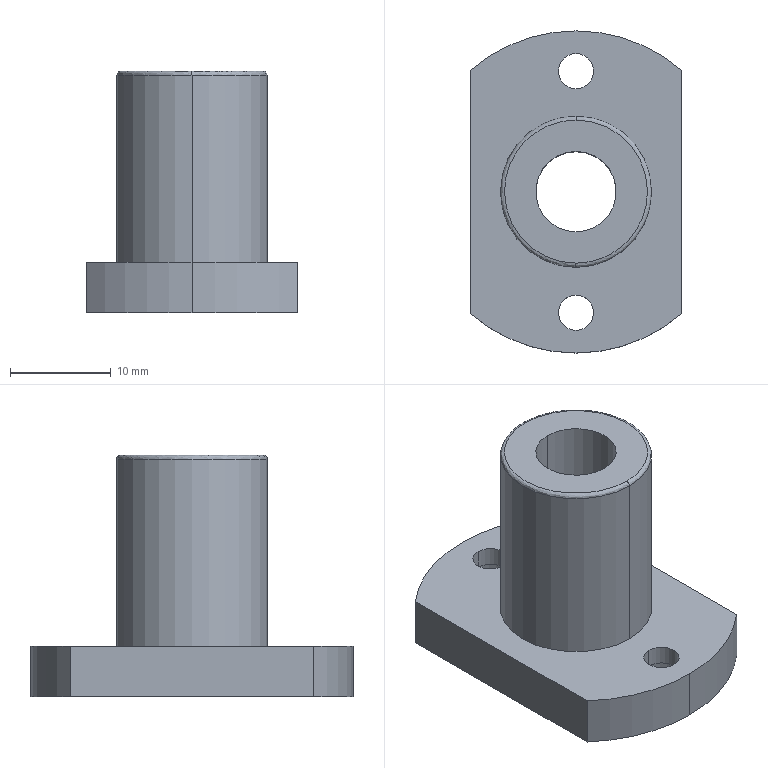Component | SolidWorks | 170423A4-LME21-d8-1 | 1 solid | 24 faces | box 21 x 32 x 24 mm | volume 5038 mm3 | cylinder 15 | plane 7 | spline 2 | commonest cylinder face diameters 3.5 x4 6 x4 32 x3 15 x2 8 x2
STEP:
#1=CARTESIAN_POINT('',(-1.745,-1.815,0.6506));
#2=VERTEX_POINT('',#1);
#3=CARTESIAN_POINT('',(-1.745,-1.225,0.6506));
#4=VERTEX_POINT('',#3);
#5=CARTESIAN_POINT('',(-1.745,-1.52,0.6506));
#6=DIRECTION('',(0.,-0.,-1.));
#7=DIRECTION('',(0.,-1.,0.));
#8=AXIS2_PLACEMENT_3D('',#5,#6,#7);
#9=CIRCLE('',#8,0.2953);
#10=EDGE_CURVE('',#2,#4,#9,.T.);
#11=ORIENTED_EDGE('',*,*,#10,.F.);
#12=CARTESIAN_POINT('',(-1.745,-1.8,0.6664));
#13=VERTEX_POINT('',#12);
#14=CARTESIAN_POINT('',(-1.745,-1.8,0.6506));
#15=DIRECTION('',(-1.,-0.,-0.));
#16=DIRECTION('',(0.,-1.,0.));
#17=AXIS2_PLACEMENT_3D('',#14,#15,#16);
#18=CIRCLE('',#17,0.01575);
#19=EDGE_CURVE('',#2,#13,#18,.T.);
#20=ORIENTED_EDGE('',*,*,#19,.T.);
#21=CARTESIAN_POINT('',(-1.745,-1.241,0.6664));
#22=VERTEX_POINT('',#21);
#23=CARTESIAN_POINT('',(-1.745,-1.8,0.6664));
#24=CARTESIAN_POINT('',(-2.304,-1.8,0.6664));
#25=CARTESIAN_POINT('',(-2.304,-1.241,0.6664));
#26=CARTESIAN_POINT('',(-1.745,-1.241,0.6664));
#27=(BOUNDED_CURVE()B_SPLINE_CURVE(3,(#23,#24,#25,#26),.UNSPECIFIED.,.F.,.F.)B_SPLINE_CURVE_WITH_KNOTS((4,4),(0.5,1.),.UNSPECIFIED.)CURVE()GEOMETRIC_REPRESENTATION_ITEM()RATIONAL_B_SPLINE_CURVE((1.,0.3333,0.3333,1.))REPRESENTATION_ITEM(''));
#28=EDGE_CURVE('',#13,#22,#27,.T.);
#29=ORIENTED_EDGE('',*,*,#28,.T.);
#30=CARTESIAN_POINT('',(-1.745,-1.241,0.6506));
#31=DIRECTION('',(1.,0.,0.));
#32=DIRECTION('',(0.,1.,0.));
#33=AXIS2_PLACEMENT_3D('',#30,#31,#32);
#34=CIRCLE('',#33,0.01575);
#35=EDGE_CURVE('',#4,#22,#34,.T.);
#36=ORIENTED_EDGE('',*,*,#35,.F.);
#37=EDGE_LOOP('',(#11,#20,#29,#36));
#38=FACE_OUTER_BOUND('',#37,.T.);
#39=CARTESIAN_POINT('',(-1.745,-1.815,0.6506));
#40=CARTESIAN_POINT('',(-2.335,-1.815,0.6506));
#41=CARTESIAN_POINT('',(-2.335,-1.225,0.6506));
#42=CARTESIAN_POINT('',(-1.745,-1.225,0.6506));
#43=CARTESIAN_POINT('',(-1.745,-1.815,0.6599));
#44=CARTESIAN_POINT('',(-2.335,-1.815,0.6599));
#45=CARTESIAN_POINT('',(-2.335,-1.225,0.6599));
#46=CARTESIAN_POINT('',(-1.745,-1.225,0.6599));
#47=CARTESIAN_POINT('',(-1.745,-1.809,0.6664));
#48=CARTESIAN_POINT('',(-2.322,-1.809,0.6664));
#49=CARTESIAN_POINT('',(-2.322,-1.231,0.6664));
#50=CARTESIAN_POINT('',(-1.745,-1.231,0.6664));
#51=CARTESIAN_POINT('',(-1.745,-1.8,0.6664));
#52=CARTESIAN_POINT('',(-2.304,-1.8,0.6664));
#53=CARTESIAN_POINT('',(-2.304,-1.241,0.6664));
#54=CARTESIAN_POINT('',(-1.745,-1.241,0.6664));
#55=(BOUNDED_SURFACE()B_SPLINE_SURFACE(3,3,((#39,#40,#41,#42),(#43,#44,#45,#46),(#47,#48,#49,#50),(#51,#52,#53,#54)),.UNSPECIFIED.,.F.,.F.,.F.)B_SPLINE_SURFACE_WITH_KNOTS((4,4),(4,4),(0.,1.),(0.,1.),.UNSPECIFIED.)GEOMETRIC_REPRESENTATION_ITEM()RATIONAL_B_SPLINE_SURFACE(((1.,0.3333,0.3333,1.),(0.8047,0.2682,0.2682,0.8047),(0.8047,0.2682,0.2682,0.8047),(1.,0.3333,0.3333,1.)))REPRESENTATION_ITEM('')SURFACE());
#56=ADVANCED_FACE('',(#38),#55,.T.);
#57=CARTESIAN_POINT('',(-1.745,-1.815,-0.08165));
#58=VERTEX_POINT('',#57);
#59=CARTESIAN_POINT('',(-1.745,-1.225,-0.08165));
#60=VERTEX_POINT('',#59);
#61=CARTESIAN_POINT('',(-1.745,-1.52,-0.08165));
#62=DIRECTION('',(-0.,0.,1.));
#63=DIRECTION('',(0.,-1.,0.));
#64=AXIS2_PLACEMENT_3D('',#61,#62,#63);
#65=CIRCLE('',#64,0.2953);
#66=EDGE_CURVE('',#58,#60,#65,.T.);
#67=ORIENTED_EDGE('',*,*,#66,.T.);
#68=CARTESIAN_POINT('',(-1.745,-1.225,-0.2785));
#69=DIRECTION('',(-0.,0.,1.));
#70=VECTOR('',#69,39.37);
#71=LINE('',#68,#70);
#72=EDGE_CURVE('',#60,#4,#71,.T.);
#73=ORIENTED_EDGE('',*,*,#72,.T.);
#74=CARTESIAN_POINT('',(-1.745,-1.52,0.6506));
#75=DIRECTION('',(0.,-0.,-1.));
#76=DIRECTION('',(0.,-1.,0.));
#77=AXIS2_PLACEMENT_3D('',#74,#75,#76);
#78=CIRCLE('',#77,0.2953);
#79=EDGE_CURVE('',#4,#2,#78,.T.);
#80=ORIENTED_EDGE('',*,*,#79,.T.);
#81=CARTESIAN_POINT('',(-1.745,-1.815,-0.2785));
#82=DIRECTION('',(-0.,0.,1.));
#83=VECTOR('',#82,39.37);
#84=LINE('',#81,#83);
#85=EDGE_CURVE('',#58,#2,#84,.T.);
#86=ORIENTED_EDGE('',*,*,#85,.F.);
#87=EDGE_LOOP('',(#67,#73,#80,#86));
#88=FACE_OUTER_BOUND('',#87,.T.);
#89=CARTESIAN_POINT('',(-1.745,-1.52,-0.2785));
#90=DIRECTION('',(-0.,0.,1.));
#91=DIRECTION('',(0.,-1.,0.));
#92=AXIS2_PLACEMENT_3D('',#89,#90,#91);
#93=CYLINDRICAL_SURFACE('',#92,0.2953);
#94=ADVANCED_FACE('',(#88),#93,.T.);
#95=CARTESIAN_POINT('',(-1.745,-2.061,-0.08165));
#96=VERTEX_POINT('',#95);
#97=CARTESIAN_POINT('',(-1.745,-1.924,-0.08165));
#98=VERTEX_POINT('',#97);
#99=CARTESIAN_POINT('',(-1.745,-1.993,-0.08165));
#100=DIRECTION('',(0.,0.,-1.));
#101=DIRECTION('',(0.,1.,-0.));
#102=AXIS2_PLACEMENT_3D('',#99,#100,#101);
#103=CIRCLE('',#102,0.0689);
#104=EDGE_CURVE('',#96,#98,#103,.T.);
#105=ORIENTED_EDGE('',*,*,#104,.F.);
#106=CARTESIAN_POINT('',(-1.745,-2.061,-0.1564));
#107=VERTEX_POINT('',#106);
#108=CARTESIAN_POINT('',(-1.745,-2.061,-0.08165));
#109=DIRECTION('',(0.,0.,-1.));
#110=VECTOR('',#109,39.37);
#111=LINE('',#108,#110);
#112=EDGE_CURVE('',#96,#107,#111,.T.);
#113=ORIENTED_EDGE('',*,*,#112,.T.);
#114=CARTESIAN_POINT('',(-1.745,-1.924,-0.1564));
#115=VERTEX_POINT('',#114);
#116=CARTESIAN_POINT('',(-1.745,-1.993,-0.1564));
#117=DIRECTION('',(-0.,-0.,1.));
#118=DIRECTION('',(0.,1.,0.));
#119=AXIS2_PLACEMENT_3D('',#116,#117,#118);
#120=CIRCLE('',#119,0.0689);
#121=EDGE_CURVE('',#115,#107,#120,.T.);
#122=ORIENTED_EDGE('',*,*,#121,.F.);
#123=CARTESIAN_POINT('',(-1.745,-1.924,-0.08165));
#124=DIRECTION('',(0.,0.,-1.));
#125=VECTOR('',#124,39.37);
#126=LINE('',#123,#125);
#127=EDGE_CURVE('',#98,#115,#126,.T.);
#128=ORIENTED_EDGE('',*,*,#127,.F.);
#129=EDGE_LOOP('',(#105,#113,#122,#128));
#130=FACE_OUTER_BOUND('',#129,.T.);
#131=CARTESIAN_POINT('',(-1.745,-1.993,-0.08165));
#132=DIRECTION('',(0.,0.,-1.));
#133=DIRECTION('',(0.,1.,-0.));
#134=AXIS2_PLACEMENT_3D('',#131,#132,#133);
#135=CYLINDRICAL_SURFACE('',#134,0.0689);
#136=ADVANCED_FACE('',(#130),#135,.F.);
#137=CARTESIAN_POINT('',(-2.158,-1.995,-0.2785));
#138=VERTEX_POINT('',#137);
#139=CARTESIAN_POINT('',(-1.745,-2.15,-0.2785));
#140=VERTEX_POINT('',#139);
#141=CARTESIAN_POINT('',(-1.745,-1.52,-0.2785));
#142=DIRECTION('',(-0.,-0.,1.));
#143=DIRECTION('',(0.,-1.,0.));
#144=AXIS2_PLACEMENT_3D('',#141,#142,#143);
#145=CIRCLE('',#144,0.6299);
#146=EDGE_CURVE('',#138,#140,#145,.T.);
#147=ORIENTED_EDGE('',*,*,#146,.T.);
#148=CARTESIAN_POINT('',(-1.745,-2.15,-0.08165));
#149=VERTEX_POINT('',#148);
#150=CARTESIAN_POINT('',(-1.745,-2.15,-0.08165));
#151=DIRECTION('',(-0.,-0.,1.));
#152=VECTOR('',#151,39.37);
#153=LINE('',#150,#152);
#154=EDGE_CURVE('',#140,#149,#153,.T.);
#155=ORIENTED_EDGE('',*,*,#154,.T.);
#156=CARTESIAN_POINT('',(-2.158,-1.995,-0.08165));
#157=VERTEX_POINT('',#156);
#158=CARTESIAN_POINT('',(-1.745,-1.52,-0.08165));
#159=DIRECTION('',(-0.,-0.,1.));
#160=DIRECTION('',(0.,-1.,0.));
#161=AXIS2_PLACEMENT_3D('',#158,#159,#160);
#162=CIRCLE('',#161,0.6299);
#163=EDGE_CURVE('',#157,#149,#162,.T.);
#164=ORIENTED_EDGE('',*,*,#163,.F.);
#165=CARTESIAN_POINT('',(-2.158,-1.995,-0.08165));
#166=DIRECTION('',(0.,0.,-1.));
#167=VECTOR('',#166,39.37);
#168=LINE('',#165,#167);
#169=EDGE_CURVE('',#157,#138,#168,.T.);
#170=ORIENTED_EDGE('',*,*,#169,.T.);
#171=EDGE_LOOP('',(#147,#155,#164,#170));
#172=FACE_OUTER_BOUND('',#171,.T.);
#173=CARTESIAN_POINT('',(-1.745,-1.52,-0.08165));
#174=DIRECTION('',(-0.,-0.,1.));
#175=DIRECTION('',(0.,-1.,0.));
#176=AXIS2_PLACEMENT_3D('',#173,#174,#175);
#177=CYLINDRICAL_SURFACE('',#176,0.6299);
#178=ADVANCED_FACE('',(#172),#177,.T.);
#179=CARTESIAN_POINT('',(-1.745,-0.9788,-0.1564));
#180=VERTEX_POINT('',#179);
#181=CARTESIAN_POINT('',(-1.745,-1.117,-0.1564));
#182=VERTEX_POINT('',#181);
#183=CARTESIAN_POINT('',(-1.745,-1.048,-0.1564));
#184=DIRECTION('',(-0.,-0.,1.));
#185=DIRECTION('',(0.,-1.,0.));
#186=AXIS2_PLACEMENT_3D('',#183,#184,#185);
#187=CIRCLE('',#186,0.0689);
#188=EDGE_CURVE('',#180,#182,#187,.T.);
#189=ORIENTED_EDGE('',*,*,#188,.F.);
#190=CARTESIAN_POINT('',(-1.745,-0.9788,-0.08165));
#191=VERTEX_POINT('',#190);
#192=CARTESIAN_POINT('',(-1.745,-0.9788,-0.2785));
#193=DIRECTION('',(-0.,-0.,1.));
#194=VECTOR('',#193,39.37);
#195=LINE('',#192,#194);
#196=EDGE_CURVE('',#180,#191,#195,.T.);
#197=ORIENTED_EDGE('',*,*,#196,.T.);
#198=CARTESIAN_POINT('',(-1.745,-1.117,-0.08165));
#199=VERTEX_POINT('',#198);
#200=CARTESIAN_POINT('',(-1.745,-1.048,-0.08165));
#201=DIRECTION('',(0.,0.,-1.));
#202=DIRECTION('',(0.,-1.,0.));
#203=AXIS2_PLACEMENT_3D('',#200,#201,#202);
#204=CIRCLE('',#203,0.0689);
#205=EDGE_CURVE('',#199,#191,#204,.T.);
#206=ORIENTED_EDGE('',*,*,#205,.F.);
#207=CARTESIAN_POINT('',(-1.745,-1.117,-0.2785));
#208=DIRECTION('',(-0.,-0.,1.));
#209=VECTOR('',#208,39.37);
#210=LINE('',#207,#209);
#211=EDGE_CURVE('',#182,#199,#210,.T.);
#212=ORIENTED_EDGE('',*,*,#211,.F.);
#213=EDGE_LOOP('',(#189,#197,#206,#212));
#214=FACE_OUTER_BOUND('',#213,.T.);
#215=CARTESIAN_POINT('',(-1.745,-1.048,-0.2785));
#216=DIRECTION('',(-0.,-0.,1.));
#217=DIRECTION('',(0.,-1.,0.));
#218=AXIS2_PLACEMENT_3D('',#215,#216,#217);
#219=CYLINDRICAL_SURFACE('',#218,0.0689);
#220=ADVANCED_FACE('',(#214),#219,.F.);
#221=CARTESIAN_POINT('',(-1.745,-1.363,-0.2785));
#222=VERTEX_POINT('',#221);
#223=CARTESIAN_POINT('',(-1.745,-1.678,-0.2785));
#224=VERTEX_POINT('',#223);
#225=CARTESIAN_POINT('',(-1.745,-1.52,-0.2785));
#226=DIRECTION('',(-0.,0.,1.));
#227=DIRECTION('',(0.,-1.,0.));
#228=AXIS2_PLACEMENT_3D('',#225,#226,#227);
#229=CIRCLE('',#228,0.1575);
#230=EDGE_CURVE('',#222,#224,#229,.T.);
#231=ORIENTED_EDGE('',*,*,#230,.F.);
#232=CARTESIAN_POINT('',(-1.745,-1.363,0.6664));
#233=VERTEX_POINT('',#232);
#234=CARTESIAN_POINT('',(-1.745,-1.363,-0.2785));
#235=DIRECTION('',(-0.,0.,1.));
#236=VECTOR('',#235,39.37);
#237=LINE('',#234,#236);
#238=EDGE_CURVE('',#222,#233,#237,.T.);
#239=ORIENTED_EDGE('',*,*,#238,.T.);
#240=CARTESIAN_POINT('',(-1.745,-1.678,0.6664));
#241=VERTEX_POINT('',#240);
#242=CARTESIAN_POINT('',(-1.745,-1.52,0.6664));
#243=DIRECTION('',(0.,-0.,-1.));
#244=DIRECTION('',(0.,-1.,0.));
#245=AXIS2_PLACEMENT_3D('',#242,#243,#244);
#246=CIRCLE('',#245,0.1575);
#247=EDGE_CURVE('',#241,#233,#246,.T.);
#248=ORIENTED_EDGE('',*,*,#247,.F.);
#249=CARTESIAN_POINT('',(-1.745,-1.678,-0.2785));
#250=DIRECTION('',(-0.,0.,1.));
#251=VECTOR('',#250,39.37);
#252=LINE('',#249,#251);
#253=EDGE_CURVE('',#224,#241,#252,.T.);
#254=ORIENTED_EDGE('',*,*,#253,.F.);
#255=EDGE_LOOP('',(#231,#239,#248,#254));
#256=FACE_OUTER_BOUND('',#255,.T.);
#257=CARTESIAN_POINT('',(-1.745,-1.52,-0.2785));
#258=DIRECTION('',(-0.,0.,1.));
#259=DIRECTION('',(0.,-1.,0.));
#260=AXIS2_PLACEMENT_3D('',#257,#258,#259);
#261=CYLINDRICAL_SURFACE('',#260,0.1575);
#262=ADVANCED_FACE('',(#256),#261,.F.);
#263=CARTESIAN_POINT('',(-1.745,-2.111,-0.1564));
#264=VERTEX_POINT('',#263);
#265=CARTESIAN_POINT('',(-1.745,-1.874,-0.1564));
#266=VERTEX_POINT('',#265);
#267=CARTESIAN_POINT('',(-1.745,-1.993,-0.1564));
#268=DIRECTION('',(0.,0.,-1.));
#269=DIRECTION('',(0.,1.,-0.));
#270=AXIS2_PLACEMENT_3D('',#267,#268,#269);
#271=CIRCLE('',#270,0.1181);
#272=EDGE_CURVE('',#264,#266,#271,.T.);
#273=ORIENTED_EDGE('',*,*,#272,.F.);
#274=CARTESIAN_POINT('',(-1.745,-2.111,-0.2785));
#275=VERTEX_POINT('',#274);
#276=CARTESIAN_POINT('',(-1.745,-2.111,-0.08165));
#277=DIRECTION('',(0.,0.,-1.));
#278=VECTOR('',#277,39.37);
#279=LINE('',#276,#278);
#280=EDGE_CURVE('',#264,#275,#279,.T.);
#281=ORIENTED_EDGE('',*,*,#280,.T.);
#282=CARTESIAN_POINT('',(-1.745,-1.874,-0.2785));
#283=VERTEX_POINT('',#282);
#284=CARTESIAN_POINT('',(-1.745,-1.993,-0.2785));
#285=DIRECTION('',(-0.,-0.,1.));
#286=DIRECTION('',(0.,1.,-0.));
#287=AXIS2_PLACEMENT_3D('',#284,#285,#286);
#288=CIRCLE('',#287,0.1181);
#289=EDGE_CURVE('',#283,#275,#288,.T.);
#290=ORIENTED_EDGE('',*,*,#289,.F.);
#291=CARTESIAN_POINT('',(-1.745,-1.874,-0.08165));
#292=DIRECTION('',(0.,0.,-1.));
#293=VECTOR('',#292,39.37);
#294=LINE('',#291,#293);
#295=EDGE_CURVE('',#266,#283,#294,.T.);
#296=ORIENTED_EDGE('',*,*,#295,.F.);
#297=EDGE_LOOP('',(#273,#281,#290,#296));
#298=FACE_OUTER_BOUND('',#297,.T.);
#299=CARTESIAN_POINT('',(-1.745,-1.993,-0.08165));
#300=DIRECTION('',(0.,0.,-1.));
#301=DIRECTION('',(0.,1.,-0.));
#302=AXIS2_PLACEMENT_3D('',#299,#300,#301);
#303=CYLINDRICAL_SURFACE('',#302,0.1181);
#304=ADVANCED_FACE('',(#298),#303,.F.);
#305=CARTESIAN_POINT('',(-1.745,-0.9296,-0.2785));
#306=VERTEX_POINT('',#305);
#307=CARTESIAN_POINT('',(-1.745,-1.166,-0.2785));
#308=VERTEX_POINT('',#307);
#309=CARTESIAN_POINT('',(-1.745,-1.048,-0.2785));
#310=DIRECTION('',(-0.,-0.,1.));
#311=DIRECTION('',(0.,-1.,0.));
#312=AXIS2_PLACEMENT_3D('',#309,#310,#311);
#313=CIRCLE('',#312,0.1181);
#314=EDGE_CURVE('',#306,#308,#313,.T.);
#315=ORIENTED_EDGE('',*,*,#314,.F.);
#316=CARTESIAN_POINT('',(-1.745,-0.9296,-0.1564));
#317=VERTEX_POINT('',#316);
#318=CARTESIAN_POINT('',(-1.745,-0.9296,-0.2785));
#319=DIRECTION('',(-0.,-0.,1.));
#320=VECTOR('',#319,39.37);
#321=LINE('',#318,#320);
#322=EDGE_CURVE('',#306,#317,#321,.T.);
#323=ORIENTED_EDGE('',*,*,#322,.T.);
#324=CARTESIAN_POINT('',(-1.745,-1.166,-0.1564));
#325=VERTEX_POINT('',#324);
#326=CARTESIAN_POINT('',(-1.745,-1.048,-0.1564));
#327=DIRECTION('',(0.,0.,-1.));
#328=DIRECTION('',(0.,-1.,0.));
#329=AXIS2_PLACEMENT_3D('',#326,#327,#328);
#330=CIRCLE('',#329,0.1181);
#331=EDGE_CURVE('',#325,#317,#330,.T.);
#332=ORIENTED_EDGE('',*,*,#331,.F.);
#333=CARTESIAN_POINT('',(-1.745,-1.166,-0.2785));
#334=DIRECTION('',(-0.,-0.,1.));
#335=VECTOR('',#334,39.37);
#336=LINE('',#333,#335);
#337=EDGE_CURVE('',#308,#325,#336,.T.);
#338=ORIENTED_EDGE('',*,*,#337,.F.);
#339=EDGE_LOOP('',(#315,#323,#332,#338));
#340=FACE_OUTER_BOUND('',#339,.T.);
#341=CARTESIAN_POINT('',(-1.745,-1.048,-0.2785));
#342=DIRECTION('',(-0.,-0.,1.));
#343=DIRECTION('',(0.,-1.,0.));
#344=AXIS2_PLACEMENT_3D('',#341,#342,#343);
#345=CYLINDRICAL_SURFACE('',#344,0.1181);
#346=ADVANCED_FACE('',(#340),#345,.F.);
#347=ORIENTED_EDGE('',*,*,#72,.F.);
#348=CARTESIAN_POINT('',(-1.745,-1.52,-0.08165));
#349=DIRECTION('',(-0.,0.,1.));
#350=DIRECTION('',(0.,-1.,0.));
#351=AXIS2_PLACEMENT_3D('',#348,#349,#350);
#352=CIRCLE('',#351,0.2953);
#353=EDGE_CURVE('',#60,#58,#352,.T.);
#354=ORIENTED_EDGE('',*,*,#353,.T.);
#355=ORIENTED_EDGE('',*,*,#85,.T.);
#356=ORIENTED_EDGE('',*,*,#10,.T.);
#357=EDGE_LOOP('',(#347,#354,#355,#356));
#358=FACE_OUTER_BOUND('',#357,.T.);
#359=CARTESIAN_POINT('',(-1.745,-1.52,-0.2785));
#360=DIRECTION('',(-0.,0.,1.));
#361=DIRECTION('',(0.,-1.,0.));
#362=AXIS2_PLACEMENT_3D('',#359,#360,#361);
#363=CYLINDRICAL_SURFACE('',#362,0.2953);
#364=ADVANCED_FACE('',(#358),#363,.T.);
#365=CARTESIAN_POINT('',(-1.745,-1.993,-0.08165));
#366=DIRECTION('',(0.,0.,-1.));
#367=DIRECTION('',(0.,1.,-0.));
#368=AXIS2_PLACEMENT_3D('',#365,#366,#367);
#369=CIRCLE('',#368,0.0689);
#370=EDGE_CURVE('',#98,#96,#369,.T.);
#371=ORIENTED_EDGE('',*,*,#370,.T.);
#372=ORIENTED_EDGE('',*,*,#104,.T.);
#373=EDGE_LOOP('',(#371,#372));
#374=FACE_BOUND('',#373,.T.);
#375=CARTESIAN_POINT('',(-2.158,-1.045,-0.08165));
#376=VERTEX_POINT('',#375);
#377=CARTESIAN_POINT('',(-2.158,-1.52,-0.08165));
#378=DIRECTION('',(0.,-1.,0.));
#379=VECTOR('',#378,39.37);
#380=LINE('',#377,#379);
#381=EDGE_CURVE('',#376,#157,#380,.T.);
#382=ORIENTED_EDGE('',*,*,#381,.T.);
#383=ORIENTED_EDGE('',*,*,#163,.T.);
#384=CARTESIAN_POINT('',(-1.331,-1.995,-0.08165));
#385=VERTEX_POINT('',#384);
#386=CARTESIAN_POINT('',(-1.745,-1.52,-0.08165));
#387=DIRECTION('',(-0.,-0.,1.));
#388=DIRECTION('',(0.,-1.,0.));
#389=AXIS2_PLACEMENT_3D('',#386,#387,#388);
#390=CIRCLE('',#389,0.6299);
#391=EDGE_CURVE('',#149,#385,#390,.T.);
#392=ORIENTED_EDGE('',*,*,#391,.T.);
#393=CARTESIAN_POINT('',(-1.331,-1.045,-0.08165));
#394=VERTEX_POINT('',#393);
#395=CARTESIAN_POINT('',(-1.331,-1.52,-0.08165));
#396=DIRECTION('',(-0.,1.,-0.));
#397=VECTOR('',#396,39.37);
#398=LINE('',#395,#397);
#399=EDGE_CURVE('',#385,#394,#398,.T.);
#400=ORIENTED_EDGE('',*,*,#399,.T.);
#401=CARTESIAN_POINT('',(-1.745,-1.52,-0.08165));
#402=DIRECTION('',(-0.,-0.,1.));
#403=DIRECTION('',(0.,-1.,0.));
#404=AXIS2_PLACEMENT_3D('',#401,#402,#403);
#405=CIRCLE('',#404,0.6299);
#406=EDGE_CURVE('',#394,#376,#405,.T.);
#407=ORIENTED_EDGE('',*,*,#406,.T.);
#408=EDGE_LOOP('',(#382,#383,#392,#400,#407));
#409=FACE_OUTER_BOUND('',#408,.T.);
#410=ORIENTED_EDGE('',*,*,#66,.F.);
#411=ORIENTED_EDGE('',*,*,#353,.F.);
#412=EDGE_LOOP('',(#410,#411));
#413=FACE_BOUND('',#412,.T.);
#414=ORIENTED_EDGE('',*,*,#205,.T.);
#415=CARTESIAN_POINT('',(-1.745,-1.048,-0.08165));
#416=DIRECTION('',(0.,0.,-1.));
#417=DIRECTION('',(0.,-1.,0.));
#418=AXIS2_PLACEMENT_3D('',#415,#416,#417);
#419=CIRCLE('',#418,0.0689);
#420=EDGE_CURVE('',#191,#199,#419,.T.);
#421=ORIENTED_EDGE('',*,*,#420,.T.);
#422=EDGE_LOOP('',(#414,#421));
#423=FACE_BOUND('',#422,.T.);
#424=CARTESIAN_POINT('',(-1.745,-1.52,-0.08165));
#425=DIRECTION('',(-0.,0.,1.));
#426=DIRECTION('',(0.,-1.,0.));
#427=AXIS2_PLACEMENT_3D('',#424,#425,#426);
#428=PLANE('',#427);
#429=ADVANCED_FACE('',(#374,#409,#413,#423),#428,.T.);
#430=ORIENTED_EDGE('',*,*,#19,.F.);
#431=ORIENTED_EDGE('',*,*,#79,.F.);
#432=ORIENTED_EDGE('',*,*,#35,.T.);
#433=CARTESIAN_POINT('',(-1.745,-1.241,0.6664));
#434=CARTESIAN_POINT('',(-1.186,-1.241,0.6664));
#435=CARTESIAN_POINT('',(-1.186,-1.8,0.6664));
#436=CARTESIAN_POINT('',(-1.745,-1.8,0.6664));
#437=(BOUNDED_CURVE()B_SPLINE_CURVE(3,(#433,#434,#435,#436),.UNSPECIFIED.,.F.,.F.)B_SPLINE_CURVE_WITH_KNOTS((4,4),(0.,0.5),.UNSPECIFIED.)CURVE()GEOMETRIC_REPRESENTATION_ITEM()RATIONAL_B_SPLINE_CURVE((1.,0.3333,0.3333,1.))REPRESENTATION_ITEM(''));
#438=EDGE_CURVE('',#22,#13,#437,.T.);
#439=ORIENTED_EDGE('',*,*,#438,.T.);
#440=EDGE_LOOP('',(#430,#431,#432,#439));
#441=FACE_OUTER_BOUND('',#440,.T.);
#442=CARTESIAN_POINT('',(-1.745,-1.225,0.6506));
#443=CARTESIAN_POINT('',(-1.154,-1.225,0.6506));
#444=CARTESIAN_POINT('',(-1.154,-1.815,0.6506));
#445=CARTESIAN_POINT('',(-1.745,-1.815,0.6506));
#446=CARTESIAN_POINT('',(-1.745,-1.225,0.6599));
#447=CARTESIAN_POINT('',(-1.154,-1.225,0.6599));
#448=CARTESIAN_POINT('',(-1.154,-1.815,0.6599));
#449=CARTESIAN_POINT('',(-1.745,-1.815,0.6599));
#450=CARTESIAN_POINT('',(-1.745,-1.231,0.6664));
#451=CARTESIAN_POINT('',(-1.167,-1.231,0.6664));
#452=CARTESIAN_POINT('',(-1.167,-1.809,0.6664));
#453=CARTESIAN_POINT('',(-1.745,-1.809,0.6664));
#454=CARTESIAN_POINT('',(-1.745,-1.241,0.6664));
#455=CARTESIAN_POINT('',(-1.186,-1.241,0.6664));
#456=CARTESIAN_POINT('',(-1.186,-1.8,0.6664));
#457=CARTESIAN_POINT('',(-1.745,-1.8,0.6664));
#458=(BOUNDED_SURFACE()B_SPLINE_SURFACE(3,3,((#442,#443,#444,#445),(#446,#447,#448,#449),(#450,#451,#452,#453),(#454,#455,#456,#457)),.UNSPECIFIED.,.F.,.F.,.F.)B_SPLINE_SURFACE_WITH_KNOTS((4,4),(4,4),(0.,1.),(0.,1.),.UNSPECIFIED.)GEOMETRIC_REPRESENTATION_ITEM()RATIONAL_B_SPLINE_SURFACE(((1.,0.3333,0.3333,1.),(0.8047,0.2682,0.2682,0.8047),(0.8047,0.2682,0.2682,0.8047),(1.,0.3333,0.3333,1.)))REPRESENTATION_ITEM('')SURFACE());
#459=ADVANCED_FACE('',(#441),#458,.T.);
#460=ORIENTED_EDGE('',*,*,#112,.F.);
#461=ORIENTED_EDGE('',*,*,#370,.F.);
#462=ORIENTED_EDGE('',*,*,#127,.T.);
#463=CARTESIAN_POINT('',(-1.745,-1.993,-0.1564));
#464=DIRECTION('',(-0.,-0.,1.));
#465=DIRECTION('',(0.,1.,0.));
#466=AXIS2_PLACEMENT_3D('',#463,#464,#465);
#467=CIRCLE('',#466,0.0689);
#468=EDGE_CURVE('',#107,#115,#467,.T.);
#469=ORIENTED_EDGE('',*,*,#468,.F.);
#470=EDGE_LOOP('',(#460,#461,#462,#469));
#471=FACE_OUTER_BOUND('',#470,.T.);
#472=CARTESIAN_POINT('',(-1.745,-1.993,-0.08165));
#473=DIRECTION('',(0.,0.,-1.));
#474=DIRECTION('',(0.,1.,-0.));
#475=AXIS2_PLACEMENT_3D('',#472,#473,#474);
#476=CYLINDRICAL_SURFACE('',#475,0.0689);
#477=ADVANCED_FACE('',(#471),#476,.F.);
#478=ORIENTED_EDGE('',*,*,#154,.F.);
#479=CARTESIAN_POINT('',(-1.331,-1.995,-0.2785));
#480=VERTEX_POINT('',#479);
#481=CARTESIAN_POINT('',(-1.745,-1.52,-0.2785));
#482=DIRECTION('',(-0.,-0.,1.));
#483=DIRECTION('',(0.,-1.,0.));
#484=AXIS2_PLACEMENT_3D('',#481,#482,#483);
#485=CIRCLE('',#484,0.6299);
#486=EDGE_CURVE('',#140,#480,#485,.T.);
#487=ORIENTED_EDGE('',*,*,#486,.T.);
#488=CARTESIAN_POINT('',(-1.331,-1.995,-0.08165));
#489=DIRECTION('',(-0.,-0.,1.));
#490=VECTOR('',#489,39.37);
#491=LINE('',#488,#490);
#492=EDGE_CURVE('',#480,#385,#491,.T.);
#493=ORIENTED_EDGE('',*,*,#492,.T.);
#494=ORIENTED_EDGE('',*,*,#391,.F.);
#495=EDGE_LOOP('',(#478,#487,#493,#494));
#496=FACE_OUTER_BOUND('',#495,.T.);
#497=CARTESIAN_POINT('',(-1.745,-1.52,-0.08165));
#498=DIRECTION('',(-0.,-0.,1.));
#499=DIRECTION('',(0.,-1.,0.));
#500=AXIS2_PLACEMENT_3D('',#497,#498,#499);
#501=CYLINDRICAL_SURFACE('',#500,0.6299);
#502=ADVANCED_FACE('',(#496),#501,.T.);
#503=ORIENTED_EDGE('',*,*,#169,.F.);
#504=ORIENTED_EDGE('',*,*,#381,.F.);
#505=CARTESIAN_POINT('',(-2.158,-1.045,-0.2785));
#506=VERTEX_POINT('',#505);
#507=CARTESIAN_POINT('',(-2.158,-1.045,-0.08165));
#508=DIRECTION('',(-0.,-0.,1.));
#509=VECTOR('',#508,39.37);
#510=LINE('',#507,#509);
#511=EDGE_CURVE('',#506,#376,#510,.T.);
#512=ORIENTED_EDGE('',*,*,#511,.F.);
#513=CARTESIAN_POINT('',(-2.158,-1.045,-0.2785));
#514=DIRECTION('',(-0.,1.,-0.));
#515=VECTOR('',#514,39.37);
#516=LINE('',#513,#515);
#517=EDGE_CURVE('',#138,#506,#516,.T.);
#518=ORIENTED_EDGE('',*,*,#517,.F.);
#519=EDGE_LOOP('',(#503,#504,#512,#518));
#520=FACE_OUTER_BOUND('',#519,.T.);
#521=CARTESIAN_POINT('',(-2.158,-1.045,-0.08165));
#522=DIRECTION('',(1.,0.,0.));
#523=DIRECTION('',(-0.,-0.,1.));
#524=AXIS2_PLACEMENT_3D('',#521,#522,#523);
#525=PLANE('',#524);
#526=ADVANCED_FACE('',(#520),#525,.F.);
#527=ORIENTED_EDGE('',*,*,#406,.F.);
#528=CARTESIAN_POINT('',(-1.331,-1.045,-0.2785));
#529=VERTEX_POINT('',#528);
#530=CARTESIAN_POINT('',(-1.331,-1.045,-0.08165));
#531=DIRECTION('',(0.,0.,-1.));
#532=VECTOR('',#531,39.37);
#533=LINE('',#530,#532);
#534=EDGE_CURVE('',#394,#529,#533,.T.);
#535=ORIENTED_EDGE('',*,*,#534,.T.);
#536=CARTESIAN_POINT('',(-1.745,-1.52,-0.2785));
#537=DIRECTION('',(-0.,-0.,1.));
#538=DIRECTION('',(0.,-1.,0.));
#539=AXIS2_PLACEMENT_3D('',#536,#537,#538);
#540=CIRCLE('',#539,0.6299);
#541=EDGE_CURVE('',#529,#506,#540,.T.);
#542=ORIENTED_EDGE('',*,*,#541,.T.);
#543=ORIENTED_EDGE('',*,*,#511,.T.);
#544=EDGE_LOOP('',(#527,#535,#542,#543));
#545=FACE_OUTER_BOUND('',#544,.T.);
#546=CARTESIAN_POINT('',(-1.745,-1.52,-0.08165));
#547=DIRECTION('',(-0.,-0.,1.));
#548=DIRECTION('',(0.,-1.,0.));
#549=AXIS2_PLACEMENT_3D('',#546,#547,#548);
#550=CYLINDRICAL_SURFACE('',#549,0.6299);
#551=ADVANCED_FACE('',(#545),#550,.T.);
#552=ORIENTED_EDGE('',*,*,#534,.F.);
#553=ORIENTED_EDGE('',*,*,#399,.F.);
#554=ORIENTED_EDGE('',*,*,#492,.F.);
#555=CARTESIAN_POINT('',(-1.331,-1.995,-0.2785));
#556=DIRECTION('',(0.,-1.,0.));
#557=VECTOR('',#556,39.37);
#558=LINE('',#555,#557);
#559=EDGE_CURVE('',#529,#480,#558,.T.);
#560=ORIENTED_EDGE('',*,*,#559,.F.);
#561=EDGE_LOOP('',(#552,#553,#554,#560));
#562=FACE_OUTER_BOUND('',#561,.T.);
#563=CARTESIAN_POINT('',(-1.331,-1.995,-0.08165));
#564=DIRECTION('',(-1.,-0.,-0.));
#565=DIRECTION('',(0.,0.,-1.));
#566=AXIS2_PLACEMENT_3D('',#563,#564,#565);
#567=PLANE('',#566);
#568=ADVANCED_FACE('',(#562),#567,.F.);
#569=ORIENTED_EDGE('',*,*,#196,.F.);
#570=CARTESIAN_POINT('',(-1.745,-1.048,-0.1564));
#571=DIRECTION('',(-0.,-0.,1.));
#572=DIRECTION('',(0.,-1.,0.));
#573=AXIS2_PLACEMENT_3D('',#570,#571,#572);
#574=CIRCLE('',#573,0.0689);
#575=EDGE_CURVE('',#182,#180,#574,.T.);
#576=ORIENTED_EDGE('',*,*,#575,.F.);
#577=ORIENTED_EDGE('',*,*,#211,.T.);
#578=ORIENTED_EDGE('',*,*,#420,.F.);
#579=EDGE_LOOP('',(#569,#576,#577,#578));
#580=FACE_OUTER_BOUND('',#579,.T.);
#581=CARTESIAN_POINT('',(-1.745,-1.048,-0.2785));
#582=DIRECTION('',(-0.,-0.,1.));
#583=DIRECTION('',(0.,-1.,0.));
#584=AXIS2_PLACEMENT_3D('',#581,#582,#583);
#585=CYLINDRICAL_SURFACE('',#584,0.0689);
#586=ADVANCED_FACE('',(#580),#585,.F.);
#587=ORIENTED_EDGE('',*,*,#438,.F.);
#588=ORIENTED_EDGE('',*,*,#28,.F.);
#589=EDGE_LOOP('',(#587,#588));
#590=FACE_OUTER_BOUND('',#589,.T.);
#591=ORIENTED_EDGE('',*,*,#247,.T.);
#592=CARTESIAN_POINT('',(-1.745,-1.52,0.6664));
#593=DIRECTION('',(0.,-0.,-1.));
#594=DIRECTION('',(0.,-1.,0.));
#595=AXIS2_PLACEMENT_3D('',#592,#593,#594);
#596=CIRCLE('',#595,0.1575);
#597=EDGE_CURVE('',#233,#241,#596,.T.);
#598=ORIENTED_EDGE('',*,*,#597,.T.);
#599=EDGE_LOOP('',(#591,#598));
#600=FACE_BOUND('',#599,.T.);
#601=CARTESIAN_POINT('',(-1.745,-1.241,0.6664));
#602=DIRECTION('',(-0.,0.,1.));
#603=DIRECTION('',(0.,-1.,0.));
#604=AXIS2_PLACEMENT_3D('',#601,#602,#603);
#605=PLANE('',#604);
#606=ADVANCED_FACE('',(#590,#600),#605,.T.);
#607=CARTESIAN_POINT('',(-1.745,-1.993,-0.1564));
#608=DIRECTION('',(0.,0.,-1.));
#609=DIRECTION('',(0.,1.,-0.));
#610=AXIS2_PLACEMENT_3D('',#607,#608,#609);
#611=CIRCLE('',#610,0.1181);
#612=EDGE_CURVE('',#266,#264,#611,.T.);
#613=ORIENTED_EDGE('',*,*,#612,.T.);
#614=ORIENTED_EDGE('',*,*,#272,.T.);
#615=EDGE_LOOP('',(#613,#614));
#616=FACE_OUTER_BOUND('',#615,.T.);
#617=ORIENTED_EDGE('',*,*,#121,.T.);
#618=ORIENTED_EDGE('',*,*,#468,.T.);
#619=EDGE_LOOP('',(#617,#618));
#620=FACE_BOUND('',#619,.T.);
#621=CARTESIAN_POINT('',(-1.745,-2.111,-0.1564));
#622=DIRECTION('',(0.,-0.,-1.));
#623=DIRECTION('',(-0.,1.,-0.));
#624=AXIS2_PLACEMENT_3D('',#621,#622,#623);
#625=PLANE('',#624);
#626=ADVANCED_FACE('',(#616,#620),#625,.T.);
#627=ORIENTED_EDGE('',*,*,#289,.T.);
#628=CARTESIAN_POINT('',(-1.745,-1.993,-0.2785));
#629=DIRECTION('',(-0.,-0.,1.));
#630=DIRECTION('',(0.,1.,-0.));
#631=AXIS2_PLACEMENT_3D('',#628,#629,#630);
#632=CIRCLE('',#631,0.1181);
#633=EDGE_CURVE('',#275,#283,#632,.T.);
#634=ORIENTED_EDGE('',*,*,#633,.T.);
#635=EDGE_LOOP('',(#627,#634));
#636=FACE_BOUND('',#635,.T.);
#637=ORIENTED_EDGE('',*,*,#517,.T.);
#638=ORIENTED_EDGE('',*,*,#541,.F.);
#639=ORIENTED_EDGE('',*,*,#559,.T.);
#640=ORIENTED_EDGE('',*,*,#486,.F.);
#641=ORIENTED_EDGE('',*,*,#146,.F.);
#642=EDGE_LOOP('',(#637,#638,#639,#640,#641));
#643=FACE_OUTER_BOUND('',#642,.T.);
#644=CARTESIAN_POINT('',(-1.745,-1.52,-0.2785));
#645=DIRECTION('',(-0.,0.,1.));
#646=DIRECTION('',(0.,-1.,0.));
#647=AXIS2_PLACEMENT_3D('',#644,#645,#646);
#648=CIRCLE('',#647,0.1575);
#649=EDGE_CURVE('',#224,#222,#648,.T.);
#650=ORIENTED_EDGE('',*,*,#649,.T.);
#651=ORIENTED_EDGE('',*,*,#230,.T.);
#652=EDGE_LOOP('',(#650,#651));
#653=FACE_BOUND('',#652,.T.);
#654=CARTESIAN_POINT('',(-1.745,-1.048,-0.2785));
#655=DIRECTION('',(-0.,-0.,1.));
#656=DIRECTION('',(0.,-1.,0.));
#657=AXIS2_PLACEMENT_3D('',#654,#655,#656);
#658=CIRCLE('',#657,0.1181);
#659=EDGE_CURVE('',#308,#306,#658,.T.);
#660=ORIENTED_EDGE('',*,*,#659,.T.);
#661=ORIENTED_EDGE('',*,*,#314,.T.);
#662=EDGE_LOOP('',(#660,#661));
#663=FACE_BOUND('',#662,.T.);
#664=CARTESIAN_POINT('',(-1.745,-1.363,-0.2785));
#665=DIRECTION('',(0.,-0.,-1.));
#666=DIRECTION('',(-0.,1.,-0.));
#667=AXIS2_PLACEMENT_3D('',#664,#665,#666);
#668=PLANE('',#667);
#669=ADVANCED_FACE('',(#636,#643,#653,#663),#668,.T.);
#670=ORIENTED_EDGE('',*,*,#575,.T.);
#671=ORIENTED_EDGE('',*,*,#188,.T.);
#672=EDGE_LOOP('',(#670,#671));
#673=FACE_BOUND('',#672,.T.);
#674=ORIENTED_EDGE('',*,*,#331,.T.);
#675=CARTESIAN_POINT('',(-1.745,-1.048,-0.1564));
#676=DIRECTION('',(0.,0.,-1.));
#677=DIRECTION('',(0.,-1.,0.));
#678=AXIS2_PLACEMENT_3D('',#675,#676,#677);
#679=CIRCLE('',#678,0.1181);
#680=EDGE_CURVE('',#317,#325,#679,.T.);
#681=ORIENTED_EDGE('',*,*,#680,.T.);
#682=EDGE_LOOP('',(#674,#681));
#683=FACE_OUTER_BOUND('',#682,.T.);
#684=CARTESIAN_POINT('',(-1.745,-0.9788,-0.1564));
#685=DIRECTION('',(0.,-0.,-1.));
#686=DIRECTION('',(-0.,1.,-0.));
#687=AXIS2_PLACEMENT_3D('',#684,#685,#686);
#688=PLANE('',#687);
#689=ADVANCED_FACE('',(#673,#683),#688,.T.);
#690=ORIENTED_EDGE('',*,*,#238,.F.);
#691=ORIENTED_EDGE('',*,*,#649,.F.);
#692=ORIENTED_EDGE('',*,*,#253,.T.);
#693=ORIENTED_EDGE('',*,*,#597,.F.);
#694=EDGE_LOOP('',(#690,#691,#692,#693));
#695=FACE_OUTER_BOUND('',#694,.T.);
#696=CARTESIAN_POINT('',(-1.745,-1.52,-0.2785));
#697=DIRECTION('',(-0.,0.,1.));
#698=DIRECTION('',(0.,-1.,0.));
#699=AXIS2_PLACEMENT_3D('',#696,#697,#698);
#700=CYLINDRICAL_SURFACE('',#699,0.1575);
#701=ADVANCED_FACE('',(#695),#700,.F.);
#702=ORIENTED_EDGE('',*,*,#280,.F.);
#703=ORIENTED_EDGE('',*,*,#612,.F.);
#704=ORIENTED_EDGE('',*,*,#295,.T.);
#705=ORIENTED_EDGE('',*,*,#633,.F.);
#706=EDGE_LOOP('',(#702,#703,#704,#705));
#707=FACE_OUTER_BOUND('',#706,.T.);
#708=CARTESIAN_POINT('',(-1.745,-1.993,-0.08165));
#709=DIRECTION('',(0.,0.,-1.));
#710=DIRECTION('',(0.,1.,-0.));
#711=AXIS2_PLACEMENT_3D('',#708,#709,#710);
#712=CYLINDRICAL_SURFACE('',#711,0.1181);
#713=ADVANCED_FACE('',(#707),#712,.F.);
#714=ORIENTED_EDGE('',*,*,#322,.F.);
#715=ORIENTED_EDGE('',*,*,#659,.F.);
#716=ORIENTED_EDGE('',*,*,#337,.T.);
#717=ORIENTED_EDGE('',*,*,#680,.F.);
#718=EDGE_LOOP('',(#714,#715,#716,#717));
#719=FACE_OUTER_BOUND('',#718,.T.);
#720=CARTESIAN_POINT('',(-1.745,-1.048,-0.2785));
#721=DIRECTION('',(-0.,-0.,1.));
#722=DIRECTION('',(0.,-1.,0.));
#723=AXIS2_PLACEMENT_3D('',#720,#721,#722);
#724=CYLINDRICAL_SURFACE('',#723,0.1181);
#725=ADVANCED_FACE('',(#719),#724,.F.);
#726=CLOSED_SHELL('',(#56,#94,#136,#178,#220,#262,#304,#346,#364,#429,#459,#477,#502,#526,#551,#568,#586,#606,#626,#669,#689,#701,#713,#725));
#727=MANIFOLD_SOLID_BREP('',#726);
#728=CARTESIAN_POINT('',(0.,0.,0.));
#729=DIRECTION('',(0.,0.,1.));
#730=DIRECTION('',(1.,0.,0.));
#731=AXIS2_PLACEMENT_3D('',#728,#729,#730);
#732=(LENGTH_UNIT()NAMED_UNIT(*)SI_UNIT($,.METRE.));
#733=LENGTH_MEASURE_WITH_UNIT(LENGTH_MEASURE(0.0254),#732);
#734=DIMENSIONAL_EXPONENTS(1.,0.,0.,0.,0.,0.,0.);
#735=(CONVERSION_BASED_UNIT('',#733)LENGTH_UNIT()NAMED_UNIT(#734));
#736=UNCERTAINTY_MEASURE_WITH_UNIT(LENGTH_MEASURE(0.00001),#735,'','');
#737=(NAMED_UNIT(*)PLANE_ANGLE_UNIT()SI_UNIT($,.RADIAN.));
#738=(NAMED_UNIT(*)SI_UNIT($,.STERADIAN.)SOLID_ANGLE_UNIT());
#739=(GEOMETRIC_REPRESENTATION_CONTEXT(3)GLOBAL_UNCERTAINTY_ASSIGNED_CONTEXT((#736))GLOBAL_UNIT_ASSIGNED_CONTEXT((#735,#737,#738))REPRESENTATION_CONTEXT('',''));
#740=ADVANCED_BREP_SHAPE_REPRESENTATION('',(#727,#731),#739);
#741=COLOUR_RGB('',0.7922,0.8196,0.9333);
#742=FILL_AREA_STYLE_COLOUR('',#741);
#743=FILL_AREA_STYLE('',(#742));
#744=SURFACE_STYLE_FILL_AREA(#743);
#745=SURFACE_SIDE_STYLE('',(#744));
#746=SURFACE_STYLE_USAGE(.BOTH.,#745);
#747=PRESENTATION_STYLE_ASSIGNMENT((#746));
#748=STYLED_ITEM('',(#747),#727);
#749=PRESENTATION_LAYER_ASSIGNMENT('','',(#748));
#750=(LENGTH_UNIT()NAMED_UNIT(*)SI_UNIT($,.METRE.));
#751=LENGTH_MEASURE_WITH_UNIT(LENGTH_MEASURE(0.0254),#750);
#752=DIMENSIONAL_EXPONENTS(1.,0.,0.,0.,0.,0.,0.);
#753=(CONVERSION_BASED_UNIT('',#751)LENGTH_UNIT()NAMED_UNIT(#752));
#754=UNCERTAINTY_MEASURE_WITH_UNIT(LENGTH_MEASURE(0.00001),#753,'','');
#755=(NAMED_UNIT(*)PLANE_ANGLE_UNIT()SI_UNIT($,.RADIAN.));
#756=(NAMED_UNIT(*)SI_UNIT($,.STERADIAN.)SOLID_ANGLE_UNIT());
#757=(GEOMETRIC_REPRESENTATION_CONTEXT(3)GLOBAL_UNCERTAINTY_ASSIGNED_CONTEXT((#754))GLOBAL_UNIT_ASSIGNED_CONTEXT((#753,#755,#756))REPRESENTATION_CONTEXT('',''));
#758=MECHANICAL_DESIGN_GEOMETRIC_PRESENTATION_REPRESENTATION('',(#748),#757);